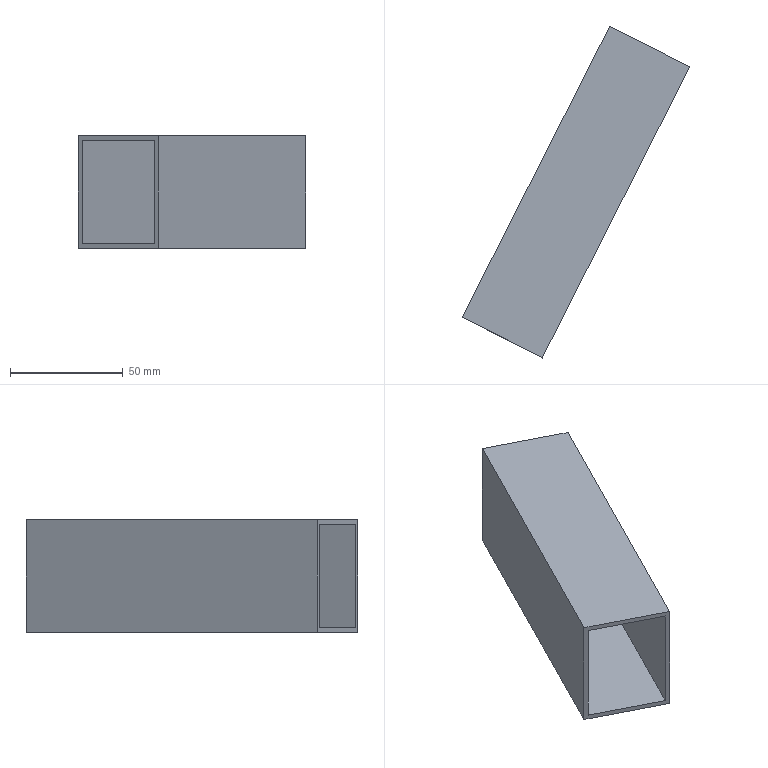Component | SolidWorks | FrameAssemblyDrawing11111-1_Part7-3 | 1 solid | 10 faces | box 101.23 x 147.42 x 50 mm | volume 49880 mm3 | plane 10
build123d program:
from build123d import *

# Parameters (mm, degrees)
SKETCH3_W           = 50
SKETCH3_H           = 145
BOSS_EXTRUDE3_DEPTH = 40
SHELL3_T            = -2


with BuildPart() as part:
    # Sketch3 → Boss-Extrude3 (new body)
    with BuildSketch(Plane.XY):
        with Locations((-63.799, 122.042)):
            Rectangle(SKETCH3_W, SKETCH3_H)
    extrude(amount=BOSS_EXTRUDE3_DEPTH)

    # Shell3
    shell3_openings = [part.faces().sort_by_distance(p)[0] for p in [
        (-63.799, 194.542, 20),
        (-63.799, 49.542, 20),
    ]]
    offset(amount=SHELL3_T, openings=shell3_openings, kind=Kind.INTERSECTION)


solid = part.part

# Placed as in the assembly
solid = solid.moved(Location((-627.944, -480.145, 1124.77), (90, 63.121, 90)))
STEP:
#1=COLOUR_RGB('',0.7922,0.8196,0.9333);
#2=FILL_AREA_STYLE_COLOUR('',#1);
#3=FILL_AREA_STYLE('',(#2));
#4=SURFACE_STYLE_FILL_AREA(#3);
#5=SURFACE_SIDE_STYLE('',(#4));
#6=SURFACE_STYLE_USAGE(.BOTH.,#5);
#7=PRESENTATION_STYLE_ASSIGNMENT((#6));
#8=CARTESIAN_POINT('',(-26.78,-26.447,40.786));
#9=VERTEX_POINT('',#8);
#10=CARTESIAN_POINT('',(-26.78,-26.447,42.755));
#11=VERTEX_POINT('',#10);
#12=CARTESIAN_POINT('',(-26.78,-26.447,40.786));
#13=DIRECTION('',(-0.,-0.,1.));
#14=VECTOR('',#13,39.37);
#15=LINE('',#12,#14);
#16=EDGE_CURVE('',#9,#11,#15,.T.);
#17=ORIENTED_EDGE('',*,*,#16,.T.);
#18=CARTESIAN_POINT('',(-28.185,-25.735,42.755));
#19=VERTEX_POINT('',#18);
#20=CARTESIAN_POINT('',(-28.185,-25.735,42.755));
#21=DIRECTION('',(0.892,-0.4521,-0.));
#22=VECTOR('',#21,39.37);
#23=LINE('',#20,#22);
#24=EDGE_CURVE('',#19,#11,#23,.T.);
#25=ORIENTED_EDGE('',*,*,#24,.F.);
#26=CARTESIAN_POINT('',(-28.185,-25.735,40.786));
#27=VERTEX_POINT('',#26);
#28=CARTESIAN_POINT('',(-28.185,-25.735,40.786));
#29=DIRECTION('',(-0.,-0.,1.));
#30=VECTOR('',#29,39.37);
#31=LINE('',#28,#30);
#32=EDGE_CURVE('',#27,#19,#31,.T.);
#33=ORIENTED_EDGE('',*,*,#32,.F.);
#34=CARTESIAN_POINT('',(-28.185,-25.735,40.786));
#35=DIRECTION('',(0.892,-0.4521,-0.));
#36=VECTOR('',#35,39.37);
#37=LINE('',#34,#36);
#38=EDGE_CURVE('',#27,#9,#37,.T.);
#39=ORIENTED_EDGE('',*,*,#38,.T.);
#40=EDGE_LOOP('',(#17,#25,#33,#39));
#41=FACE_OUTER_BOUND('',#40,.T.);
#42=CARTESIAN_POINT('',(-26.85,-26.411,40.865));
#43=VERTEX_POINT('',#42);
#44=CARTESIAN_POINT('',(-26.85,-26.411,42.676));
#45=VERTEX_POINT('',#44);
#46=CARTESIAN_POINT('',(-26.85,-26.411,40.786));
#47=DIRECTION('',(-0.,-0.,1.));
#48=VECTOR('',#47,39.37);
#49=LINE('',#46,#48);
#50=EDGE_CURVE('',#43,#45,#49,.T.);
#51=ORIENTED_EDGE('',*,*,#50,.F.);
#52=CARTESIAN_POINT('',(-28.115,-25.771,40.865));
#53=VERTEX_POINT('',#52);
#54=CARTESIAN_POINT('',(-28.185,-25.735,40.865));
#55=DIRECTION('',(0.892,-0.4521,-0.));
#56=VECTOR('',#55,39.37);
#57=LINE('',#54,#56);
#58=EDGE_CURVE('',#53,#43,#57,.T.);
#59=ORIENTED_EDGE('',*,*,#58,.F.);
#60=CARTESIAN_POINT('',(-28.115,-25.771,42.676));
#61=VERTEX_POINT('',#60);
#62=CARTESIAN_POINT('',(-28.115,-25.771,40.786));
#63=DIRECTION('',(-0.,-0.,1.));
#64=VECTOR('',#63,39.37);
#65=LINE('',#62,#64);
#66=EDGE_CURVE('',#53,#61,#65,.T.);
#67=ORIENTED_EDGE('',*,*,#66,.T.);
#68=CARTESIAN_POINT('',(-28.185,-25.735,42.676));
#69=DIRECTION('',(0.892,-0.4521,-0.));
#70=VECTOR('',#69,39.37);
#71=LINE('',#68,#70);
#72=EDGE_CURVE('',#61,#45,#71,.T.);
#73=ORIENTED_EDGE('',*,*,#72,.T.);
#74=EDGE_LOOP('',(#51,#59,#67,#73));
#75=FACE_BOUND('',#74,.T.);
#76=CARTESIAN_POINT('',(-28.185,-25.735,40.786));
#77=DIRECTION('',(0.4521,0.892,0.));
#78=DIRECTION('',(-0.892,0.4521,0.));
#79=AXIS2_PLACEMENT_3D('',#76,#77,#78);
#80=PLANE('',#79);
#81=ADVANCED_FACE('',(#41,#75),#80,.F.);
#82=CARTESIAN_POINT('',(-24.199,-21.355,42.755));
#83=VERTEX_POINT('',#82);
#84=CARTESIAN_POINT('',(-24.199,-21.355,40.786));
#85=VERTEX_POINT('',#84);
#86=CARTESIAN_POINT('',(-24.199,-21.355,40.786));
#87=DIRECTION('',(0.,0.,-1.));
#88=VECTOR('',#87,39.37);
#89=LINE('',#86,#88);
#90=EDGE_CURVE('',#83,#85,#89,.T.);
#91=ORIENTED_EDGE('',*,*,#90,.T.);
#92=CARTESIAN_POINT('',(-25.604,-20.643,40.786));
#93=VERTEX_POINT('',#92);
#94=CARTESIAN_POINT('',(-25.604,-20.643,40.786));
#95=DIRECTION('',(0.892,-0.4521,-0.));
#96=VECTOR('',#95,39.37);
#97=LINE('',#94,#96);
#98=EDGE_CURVE('',#93,#85,#97,.T.);
#99=ORIENTED_EDGE('',*,*,#98,.F.);
#100=CARTESIAN_POINT('',(-25.604,-20.643,42.755));
#101=VERTEX_POINT('',#100);
#102=CARTESIAN_POINT('',(-25.604,-20.643,40.786));
#103=DIRECTION('',(0.,0.,-1.));
#104=VECTOR('',#103,39.37);
#105=LINE('',#102,#104);
#106=EDGE_CURVE('',#101,#93,#105,.T.);
#107=ORIENTED_EDGE('',*,*,#106,.F.);
#108=CARTESIAN_POINT('',(-25.604,-20.643,42.755));
#109=DIRECTION('',(0.892,-0.4521,-0.));
#110=VECTOR('',#109,39.37);
#111=LINE('',#108,#110);
#112=EDGE_CURVE('',#101,#83,#111,.T.);
#113=ORIENTED_EDGE('',*,*,#112,.T.);
#114=EDGE_LOOP('',(#91,#99,#107,#113));
#115=FACE_OUTER_BOUND('',#114,.T.);
#116=CARTESIAN_POINT('',(-24.27,-21.319,42.676));
#117=VERTEX_POINT('',#116);
#118=CARTESIAN_POINT('',(-24.27,-21.319,40.865));
#119=VERTEX_POINT('',#118);
#120=CARTESIAN_POINT('',(-24.27,-21.319,40.786));
#121=DIRECTION('',(0.,0.,-1.));
#122=VECTOR('',#121,39.37);
#123=LINE('',#120,#122);
#124=EDGE_CURVE('',#117,#119,#123,.T.);
#125=ORIENTED_EDGE('',*,*,#124,.F.);
#126=CARTESIAN_POINT('',(-25.534,-20.679,42.676));
#127=VERTEX_POINT('',#126);
#128=CARTESIAN_POINT('',(-25.604,-20.643,42.676));
#129=DIRECTION('',(0.892,-0.4521,-0.));
#130=VECTOR('',#129,39.37);
#131=LINE('',#128,#130);
#132=EDGE_CURVE('',#127,#117,#131,.T.);
#133=ORIENTED_EDGE('',*,*,#132,.F.);
#134=CARTESIAN_POINT('',(-25.534,-20.679,40.865));
#135=VERTEX_POINT('',#134);
#136=CARTESIAN_POINT('',(-25.534,-20.679,40.786));
#137=DIRECTION('',(0.,0.,-1.));
#138=VECTOR('',#137,39.37);
#139=LINE('',#136,#138);
#140=EDGE_CURVE('',#127,#135,#139,.T.);
#141=ORIENTED_EDGE('',*,*,#140,.T.);
#142=CARTESIAN_POINT('',(-25.604,-20.643,40.865));
#143=DIRECTION('',(0.892,-0.4521,-0.));
#144=VECTOR('',#143,39.37);
#145=LINE('',#142,#144);
#146=EDGE_CURVE('',#135,#119,#145,.T.);
#147=ORIENTED_EDGE('',*,*,#146,.T.);
#148=EDGE_LOOP('',(#125,#133,#141,#147));
#149=FACE_BOUND('',#148,.T.);
#150=CARTESIAN_POINT('',(-25.604,-20.643,40.786));
#151=DIRECTION('',(-0.4521,-0.892,-0.));
#152=DIRECTION('',(0.892,-0.4521,-0.));
#153=AXIS2_PLACEMENT_3D('',#150,#151,#152);
#154=PLANE('',#153);
#155=ADVANCED_FACE('',(#115,#149),#154,.F.);
#156=CARTESIAN_POINT('',(-24.199,-21.355,40.786));
#157=DIRECTION('',(-0.4521,-0.892,-0.));
#158=VECTOR('',#157,39.37);
#159=LINE('',#156,#158);
#160=EDGE_CURVE('',#85,#9,#159,.T.);
#161=ORIENTED_EDGE('',*,*,#160,.T.);
#162=ORIENTED_EDGE('',*,*,#38,.F.);
#163=CARTESIAN_POINT('',(-25.604,-20.643,40.786));
#164=DIRECTION('',(-0.4521,-0.892,-0.));
#165=VECTOR('',#164,39.37);
#166=LINE('',#163,#165);
#167=EDGE_CURVE('',#93,#27,#166,.T.);
#168=ORIENTED_EDGE('',*,*,#167,.F.);
#169=ORIENTED_EDGE('',*,*,#98,.T.);
#170=EDGE_LOOP('',(#161,#162,#168,#169));
#171=FACE_OUTER_BOUND('',#170,.T.);
#172=CARTESIAN_POINT('',(-25.604,-20.643,40.786));
#173=DIRECTION('',(-0.,-0.,1.));
#174=DIRECTION('',(0.4521,0.892,0.));
#175=AXIS2_PLACEMENT_3D('',#172,#173,#174);
#176=PLANE('',#175);
#177=ADVANCED_FACE('',(#171),#176,.F.);
#178=CARTESIAN_POINT('',(-24.199,-21.355,42.755));
#179=DIRECTION('',(0.4521,0.892,0.));
#180=VECTOR('',#179,39.37);
#181=LINE('',#178,#180);
#182=EDGE_CURVE('',#11,#83,#181,.T.);
#183=ORIENTED_EDGE('',*,*,#182,.T.);
#184=ORIENTED_EDGE('',*,*,#112,.F.);
#185=CARTESIAN_POINT('',(-25.604,-20.643,42.755));
#186=DIRECTION('',(0.4521,0.892,0.));
#187=VECTOR('',#186,39.37);
#188=LINE('',#185,#187);
#189=EDGE_CURVE('',#19,#101,#188,.T.);
#190=ORIENTED_EDGE('',*,*,#189,.F.);
#191=ORIENTED_EDGE('',*,*,#24,.T.);
#192=EDGE_LOOP('',(#183,#184,#190,#191));
#193=FACE_OUTER_BOUND('',#192,.T.);
#194=CARTESIAN_POINT('',(-25.604,-20.643,42.755));
#195=DIRECTION('',(0.,0.,-1.));
#196=DIRECTION('',(-0.4521,-0.892,-0.));
#197=AXIS2_PLACEMENT_3D('',#194,#195,#196);
#198=PLANE('',#197);
#199=ADVANCED_FACE('',(#193),#198,.F.);
#200=ORIENTED_EDGE('',*,*,#167,.T.);
#201=ORIENTED_EDGE('',*,*,#32,.T.);
#202=ORIENTED_EDGE('',*,*,#189,.T.);
#203=ORIENTED_EDGE('',*,*,#106,.T.);
#204=EDGE_LOOP('',(#200,#201,#202,#203));
#205=FACE_OUTER_BOUND('',#204,.T.);
#206=CARTESIAN_POINT('',(-29.067,-27.475,44.282));
#207=DIRECTION('',(-0.892,0.4521,0.));
#208=DIRECTION('',(-0.,-0.,1.));
#209=AXIS2_PLACEMENT_3D('',#206,#207,#208);
#210=PLANE('',#209);
#211=ADVANCED_FACE('',(#205),#210,.T.);
#212=ORIENTED_EDGE('',*,*,#160,.F.);
#213=ORIENTED_EDGE('',*,*,#90,.F.);
#214=ORIENTED_EDGE('',*,*,#182,.F.);
#215=ORIENTED_EDGE('',*,*,#16,.F.);
#216=EDGE_LOOP('',(#212,#213,#214,#215));
#217=FACE_OUTER_BOUND('',#216,.T.);
#218=CARTESIAN_POINT('',(-27.662,-28.187,44.282));
#219=DIRECTION('',(-0.892,0.4521,0.));
#220=DIRECTION('',(-0.,-0.,1.));
#221=AXIS2_PLACEMENT_3D('',#218,#219,#220);
#222=PLANE('',#221);
#223=ADVANCED_FACE('',(#217),#222,.F.);
#224=CARTESIAN_POINT('',(-24.27,-21.319,40.865));
#225=DIRECTION('',(-0.4521,-0.892,-0.));
#226=VECTOR('',#225,39.37);
#227=LINE('',#224,#226);
#228=EDGE_CURVE('',#119,#43,#227,.T.);
#229=ORIENTED_EDGE('',*,*,#228,.F.);
#230=ORIENTED_EDGE('',*,*,#146,.F.);
#231=CARTESIAN_POINT('',(-25.534,-20.679,40.865));
#232=DIRECTION('',(-0.4521,-0.892,-0.));
#233=VECTOR('',#232,39.37);
#234=LINE('',#231,#233);
#235=EDGE_CURVE('',#135,#53,#234,.T.);
#236=ORIENTED_EDGE('',*,*,#235,.T.);
#237=ORIENTED_EDGE('',*,*,#58,.T.);
#238=EDGE_LOOP('',(#229,#230,#236,#237));
#239=FACE_OUTER_BOUND('',#238,.T.);
#240=CARTESIAN_POINT('',(-25.604,-20.643,40.865));
#241=DIRECTION('',(-0.,-0.,1.));
#242=DIRECTION('',(0.4521,0.892,0.));
#243=AXIS2_PLACEMENT_3D('',#240,#241,#242);
#244=PLANE('',#243);
#245=ADVANCED_FACE('',(#239),#244,.T.);
#246=CARTESIAN_POINT('',(-24.27,-21.319,42.676));
#247=DIRECTION('',(0.4521,0.892,0.));
#248=VECTOR('',#247,39.37);
#249=LINE('',#246,#248);
#250=EDGE_CURVE('',#45,#117,#249,.T.);
#251=ORIENTED_EDGE('',*,*,#250,.F.);
#252=ORIENTED_EDGE('',*,*,#72,.F.);
#253=CARTESIAN_POINT('',(-25.534,-20.679,42.676));
#254=DIRECTION('',(0.4521,0.892,0.));
#255=VECTOR('',#254,39.37);
#256=LINE('',#253,#255);
#257=EDGE_CURVE('',#61,#127,#256,.T.);
#258=ORIENTED_EDGE('',*,*,#257,.T.);
#259=ORIENTED_EDGE('',*,*,#132,.T.);
#260=EDGE_LOOP('',(#251,#252,#258,#259));
#261=FACE_OUTER_BOUND('',#260,.T.);
#262=CARTESIAN_POINT('',(-25.604,-20.643,42.676));
#263=DIRECTION('',(0.,0.,-1.));
#264=DIRECTION('',(-0.4521,-0.892,-0.));
#265=AXIS2_PLACEMENT_3D('',#262,#263,#264);
#266=PLANE('',#265);
#267=ADVANCED_FACE('',(#261),#266,.T.);
#268=ORIENTED_EDGE('',*,*,#235,.F.);
#269=ORIENTED_EDGE('',*,*,#140,.F.);
#270=ORIENTED_EDGE('',*,*,#257,.F.);
#271=ORIENTED_EDGE('',*,*,#66,.F.);
#272=EDGE_LOOP('',(#268,#269,#270,#271));
#273=FACE_OUTER_BOUND('',#272,.T.);
#274=CARTESIAN_POINT('',(-28.996,-27.51,44.282));
#275=DIRECTION('',(-0.892,0.4521,0.));
#276=DIRECTION('',(-0.,-0.,1.));
#277=AXIS2_PLACEMENT_3D('',#274,#275,#276);
#278=PLANE('',#277);
#279=ADVANCED_FACE('',(#273),#278,.F.);
#280=ORIENTED_EDGE('',*,*,#228,.T.);
#281=ORIENTED_EDGE('',*,*,#50,.T.);
#282=ORIENTED_EDGE('',*,*,#250,.T.);
#283=ORIENTED_EDGE('',*,*,#124,.T.);
#284=EDGE_LOOP('',(#280,#281,#282,#283));
#285=FACE_OUTER_BOUND('',#284,.T.);
#286=CARTESIAN_POINT('',(-27.732,-28.151,44.282));
#287=DIRECTION('',(-0.892,0.4521,0.));
#288=DIRECTION('',(-0.,-0.,1.));
#289=AXIS2_PLACEMENT_3D('',#286,#287,#288);
#290=PLANE('',#289);
#291=ADVANCED_FACE('',(#285),#290,.T.);
#292=CLOSED_SHELL('',(#81,#155,#177,#199,#211,#223,#245,#267,#279,#291));
#293=MANIFOLD_SOLID_BREP('',#292);
#294=STYLED_ITEM('',(#7),#293);
#295=PRESENTATION_LAYER_ASSIGNMENT('','',(#294));
#296=(LENGTH_UNIT()NAMED_UNIT(*)SI_UNIT($,.METRE.));
#297=LENGTH_MEASURE_WITH_UNIT(LENGTH_MEASURE(0.0254),#296);
#298=DIMENSIONAL_EXPONENTS(1.,0.,0.,0.,0.,0.,0.);
#299=(CONVERSION_BASED_UNIT('',#297)LENGTH_UNIT()NAMED_UNIT(#298));
#300=UNCERTAINTY_MEASURE_WITH_UNIT(LENGTH_MEASURE(0.00001),#299,'','');
#301=(NAMED_UNIT(*)PLANE_ANGLE_UNIT()SI_UNIT($,.RADIAN.));
#302=(NAMED_UNIT(*)SI_UNIT($,.STERADIAN.)SOLID_ANGLE_UNIT());
#303=(GEOMETRIC_REPRESENTATION_CONTEXT(3)GLOBAL_UNCERTAINTY_ASSIGNED_CONTEXT((#300))GLOBAL_UNIT_ASSIGNED_CONTEXT((#299,#301,#302))REPRESENTATION_CONTEXT('',''));
#304=MECHANICAL_DESIGN_GEOMETRIC_PRESENTATION_REPRESENTATION('',(#294),#303);
#305=CARTESIAN_POINT('',(0.,0.,0.));
#306=DIRECTION('',(0.,0.,1.));
#307=DIRECTION('',(1.,0.,0.));
#308=AXIS2_PLACEMENT_3D('',#305,#306,#307);
#309=(LENGTH_UNIT()NAMED_UNIT(*)SI_UNIT($,.METRE.));
#310=LENGTH_MEASURE_WITH_UNIT(LENGTH_MEASURE(0.0254),#309);
#311=DIMENSIONAL_EXPONENTS(1.,0.,0.,0.,0.,0.,0.);
#312=(CONVERSION_BASED_UNIT('',#310)LENGTH_UNIT()NAMED_UNIT(#311));
#313=UNCERTAINTY_MEASURE_WITH_UNIT(LENGTH_MEASURE(0.00001),#312,'','');
#314=(NAMED_UNIT(*)PLANE_ANGLE_UNIT()SI_UNIT($,.RADIAN.));
#315=(NAMED_UNIT(*)SI_UNIT($,.STERADIAN.)SOLID_ANGLE_UNIT());
#316=(GEOMETRIC_REPRESENTATION_CONTEXT(3)GLOBAL_UNCERTAINTY_ASSIGNED_CONTEXT((#313))GLOBAL_UNIT_ASSIGNED_CONTEXT((#312,#314,#315))REPRESENTATION_CONTEXT('',''));
#317=ADVANCED_BREP_SHAPE_REPRESENTATION('',(#293,#308),#316);